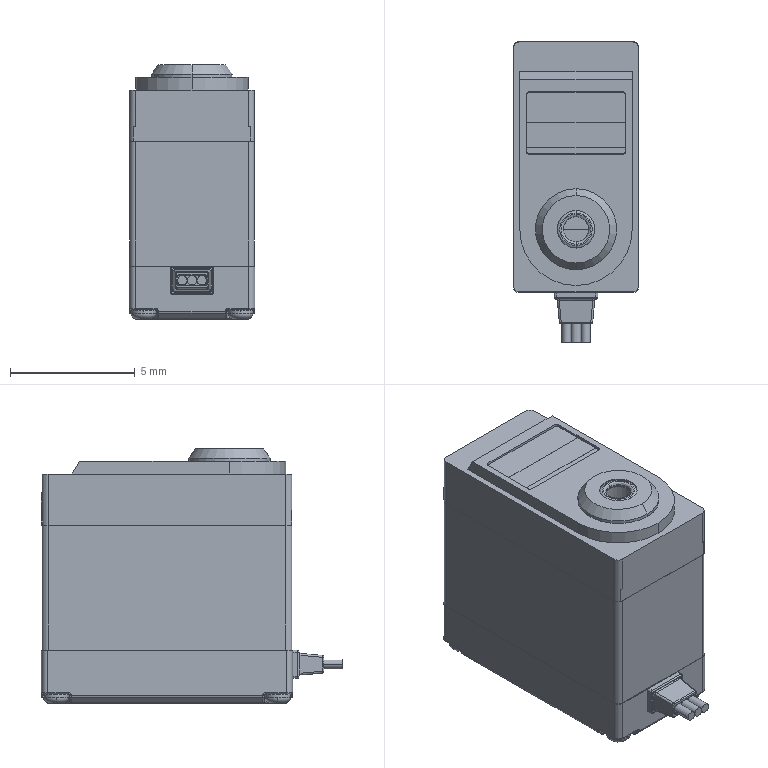Component | SolidWorks | MG996RServo_stp-4 | 10 solids | 414 faces | volume 397 mm3 | plane 177 | cylinder 149 | spline 74 | torus 12 | cone 2 | commonest cylinder face diameters 0.1 x52 0.5 x36 0.25 x16 1 x10 0.15 x8 0.375 x6 0.05 x5 1.5 x4 | material 45